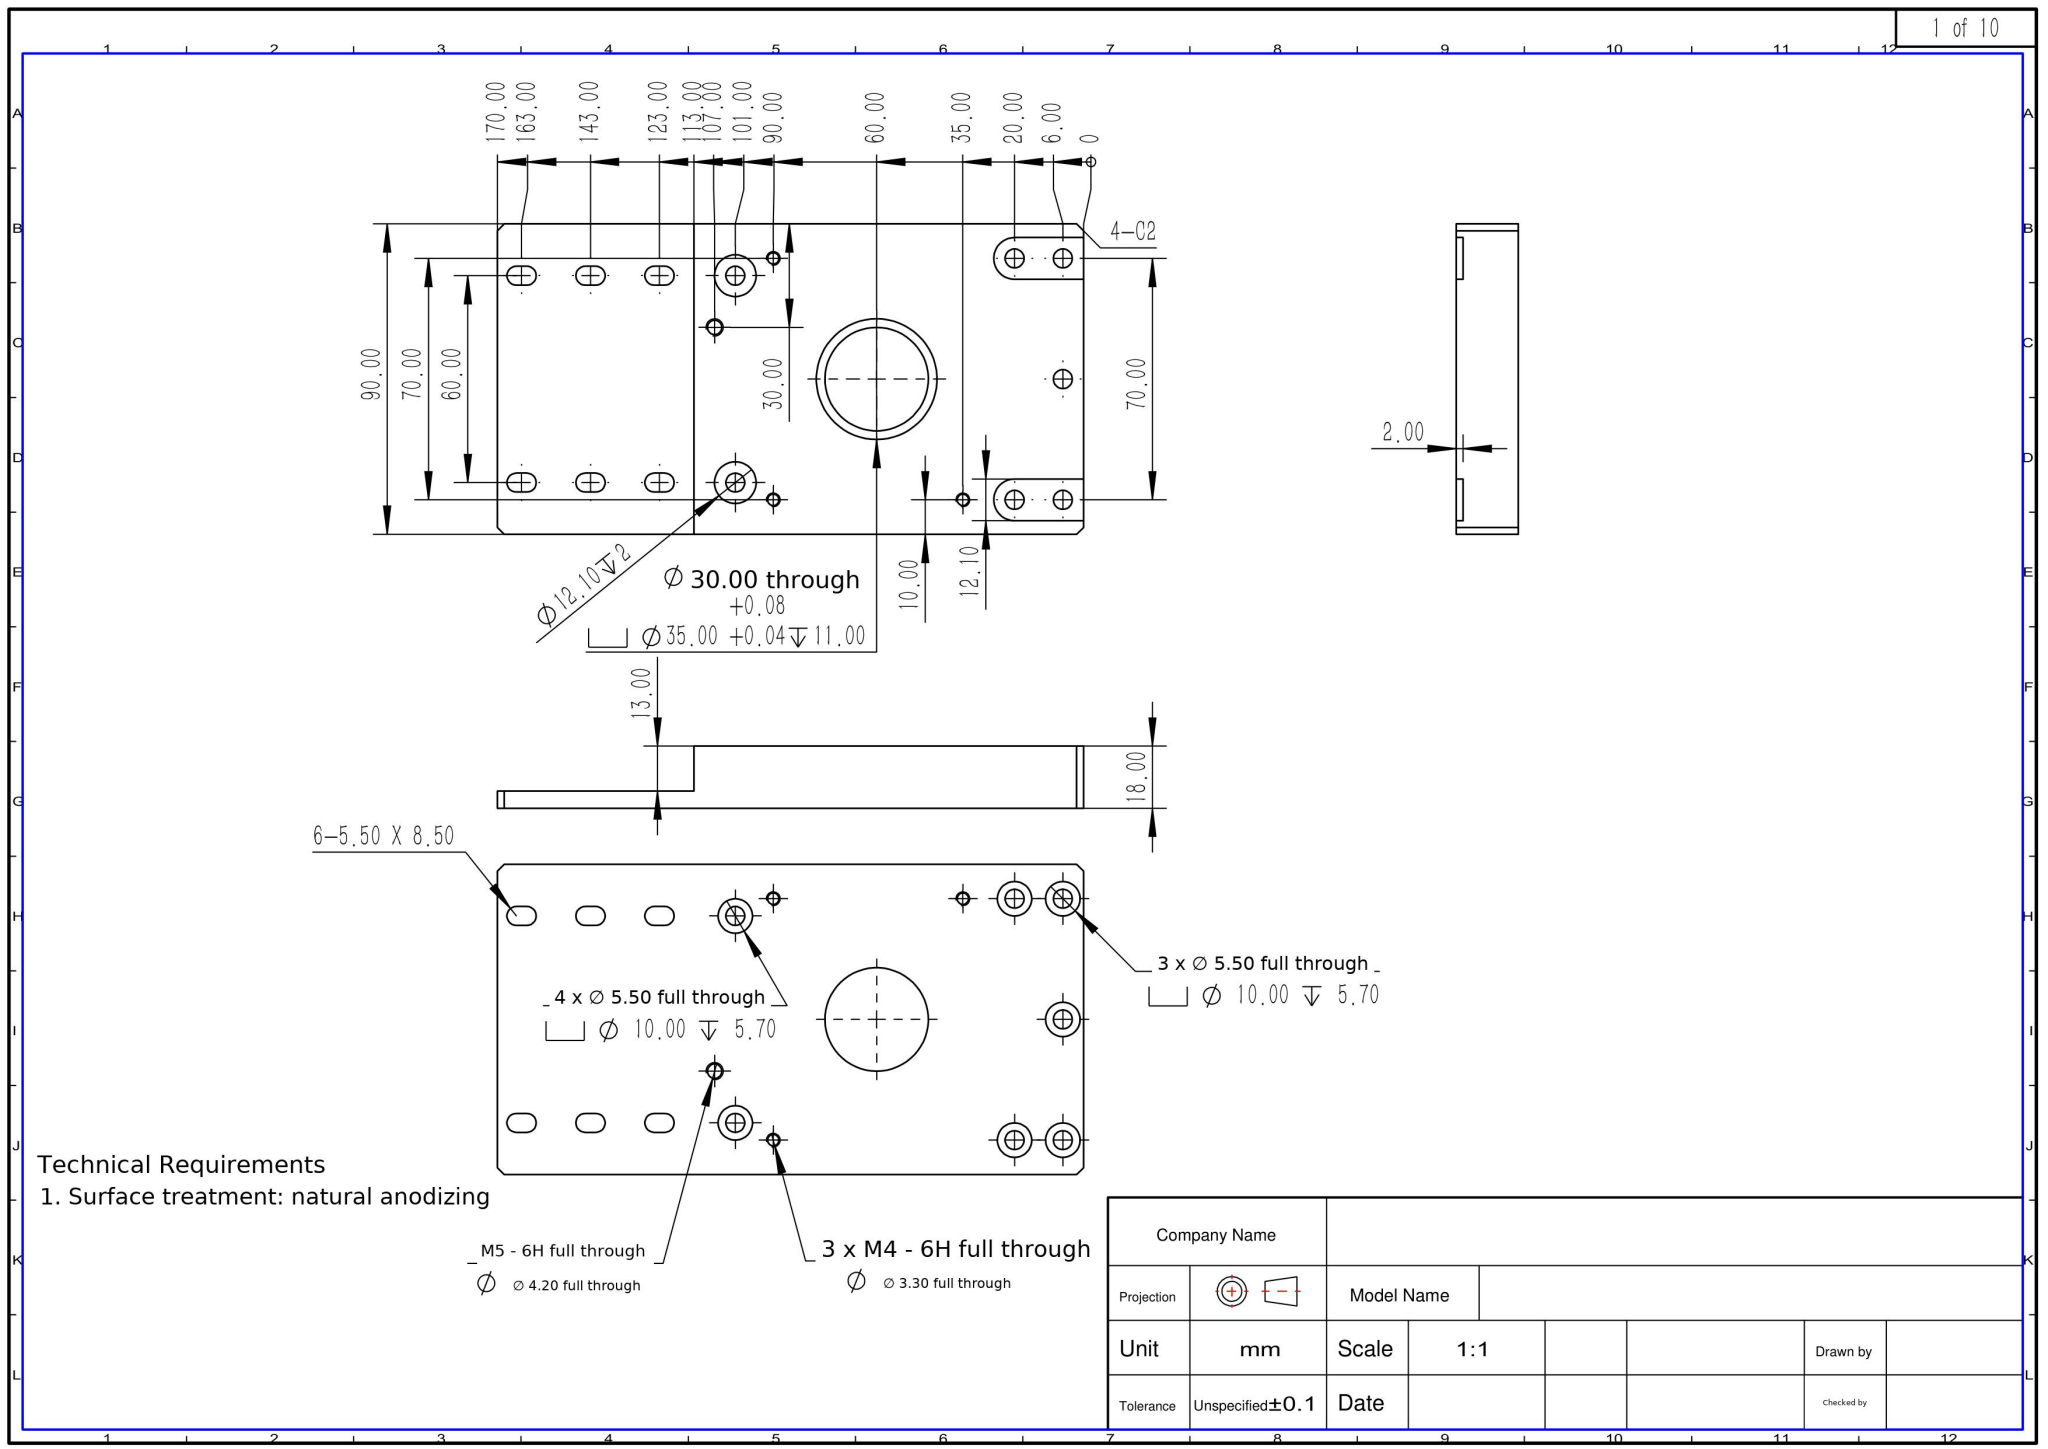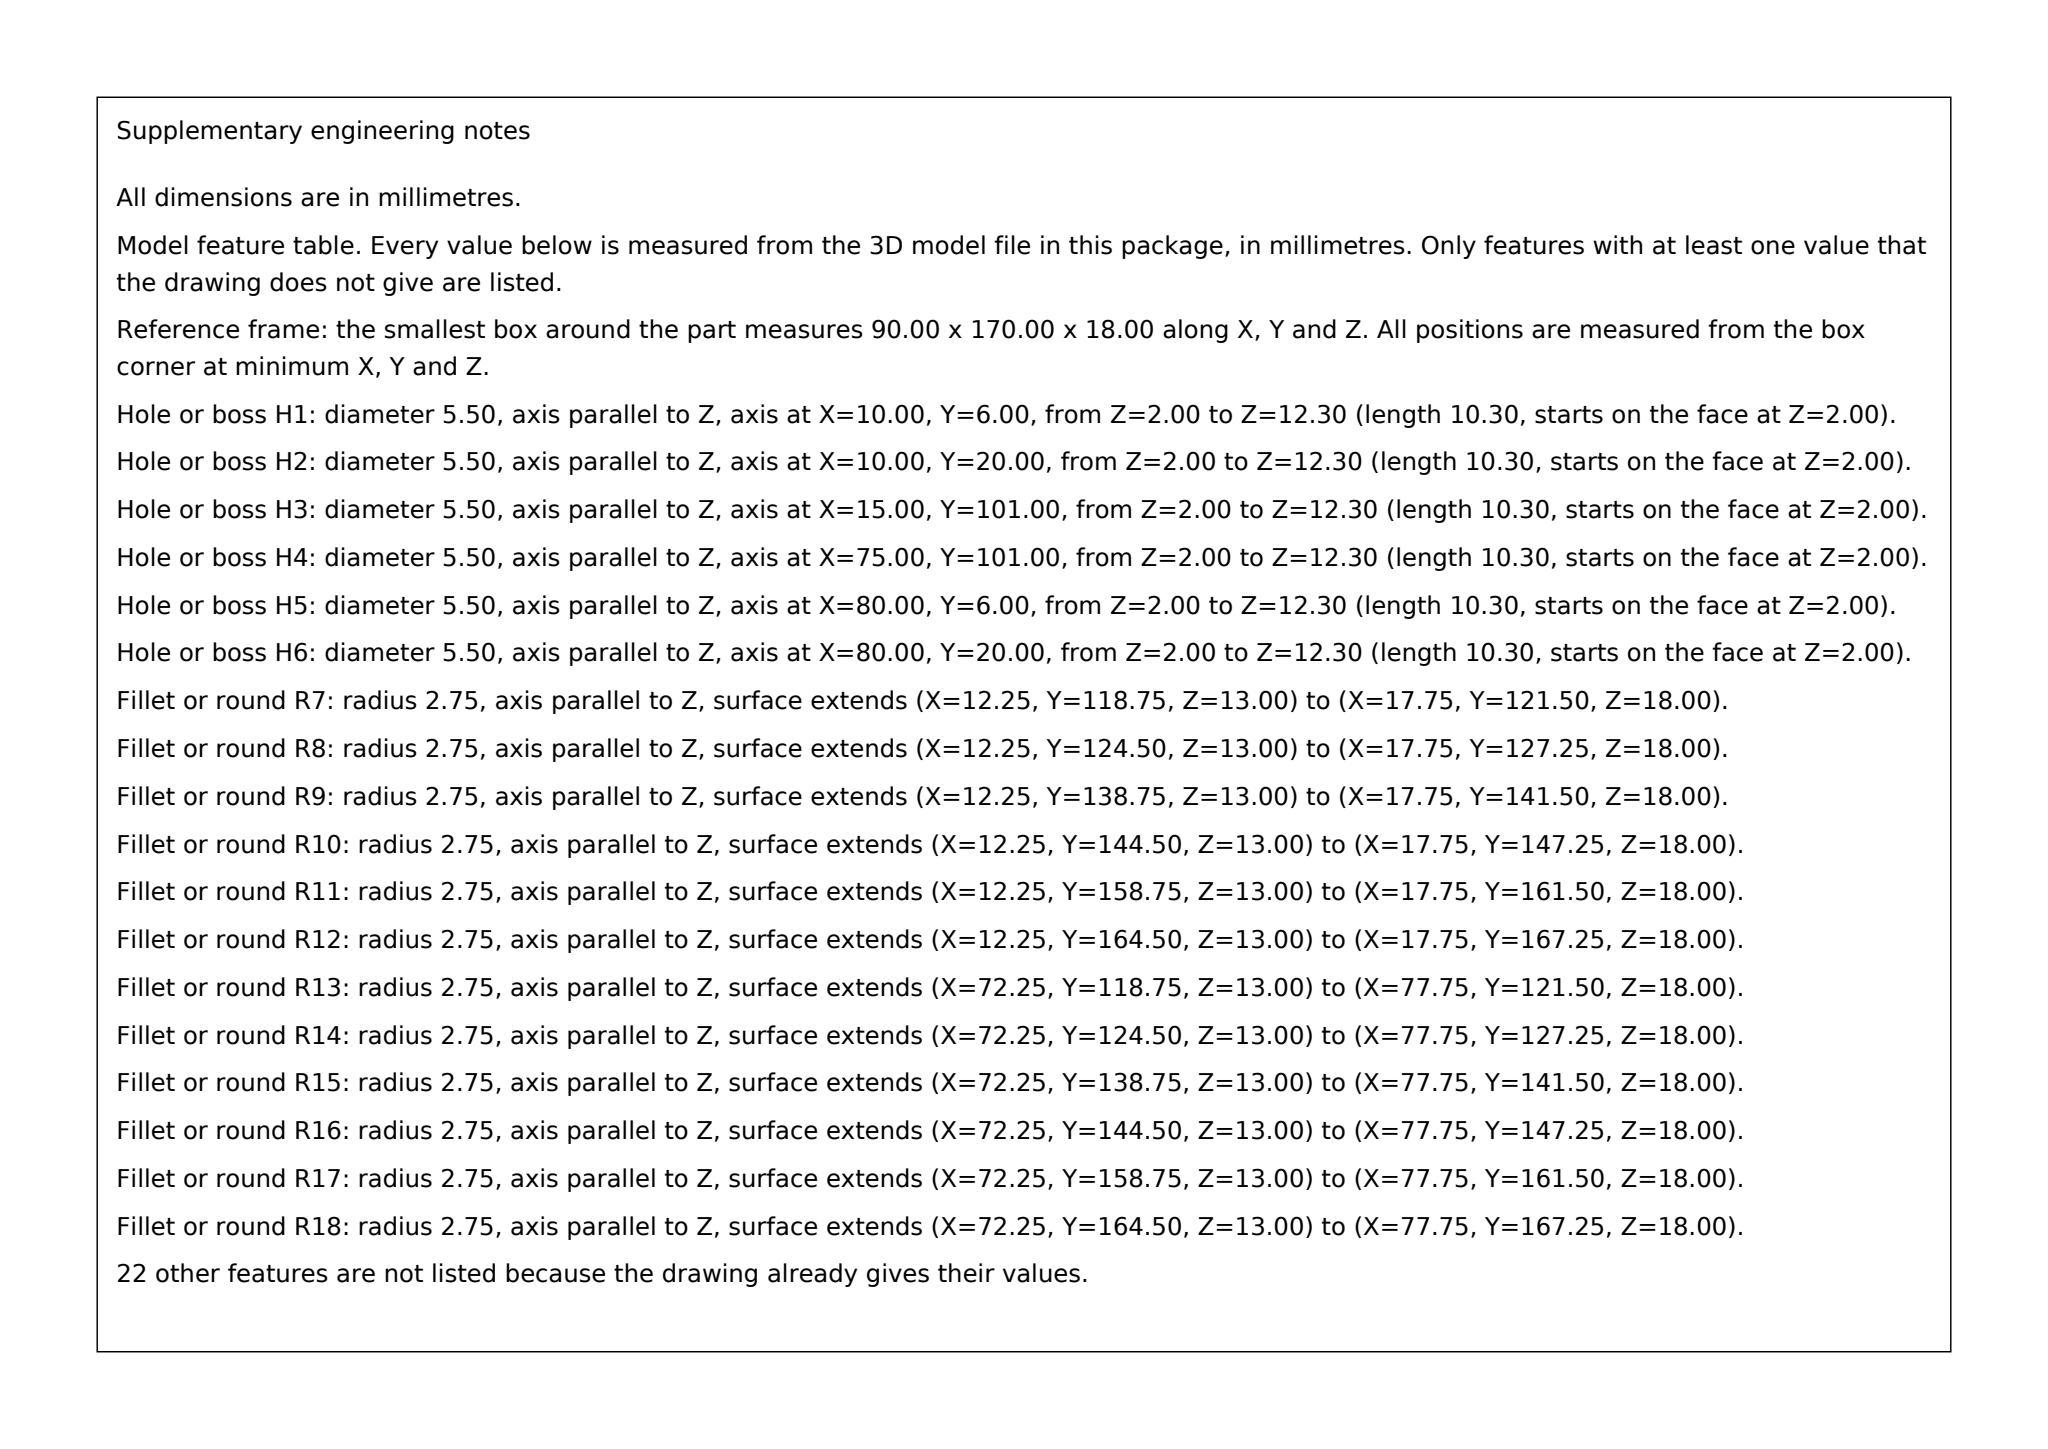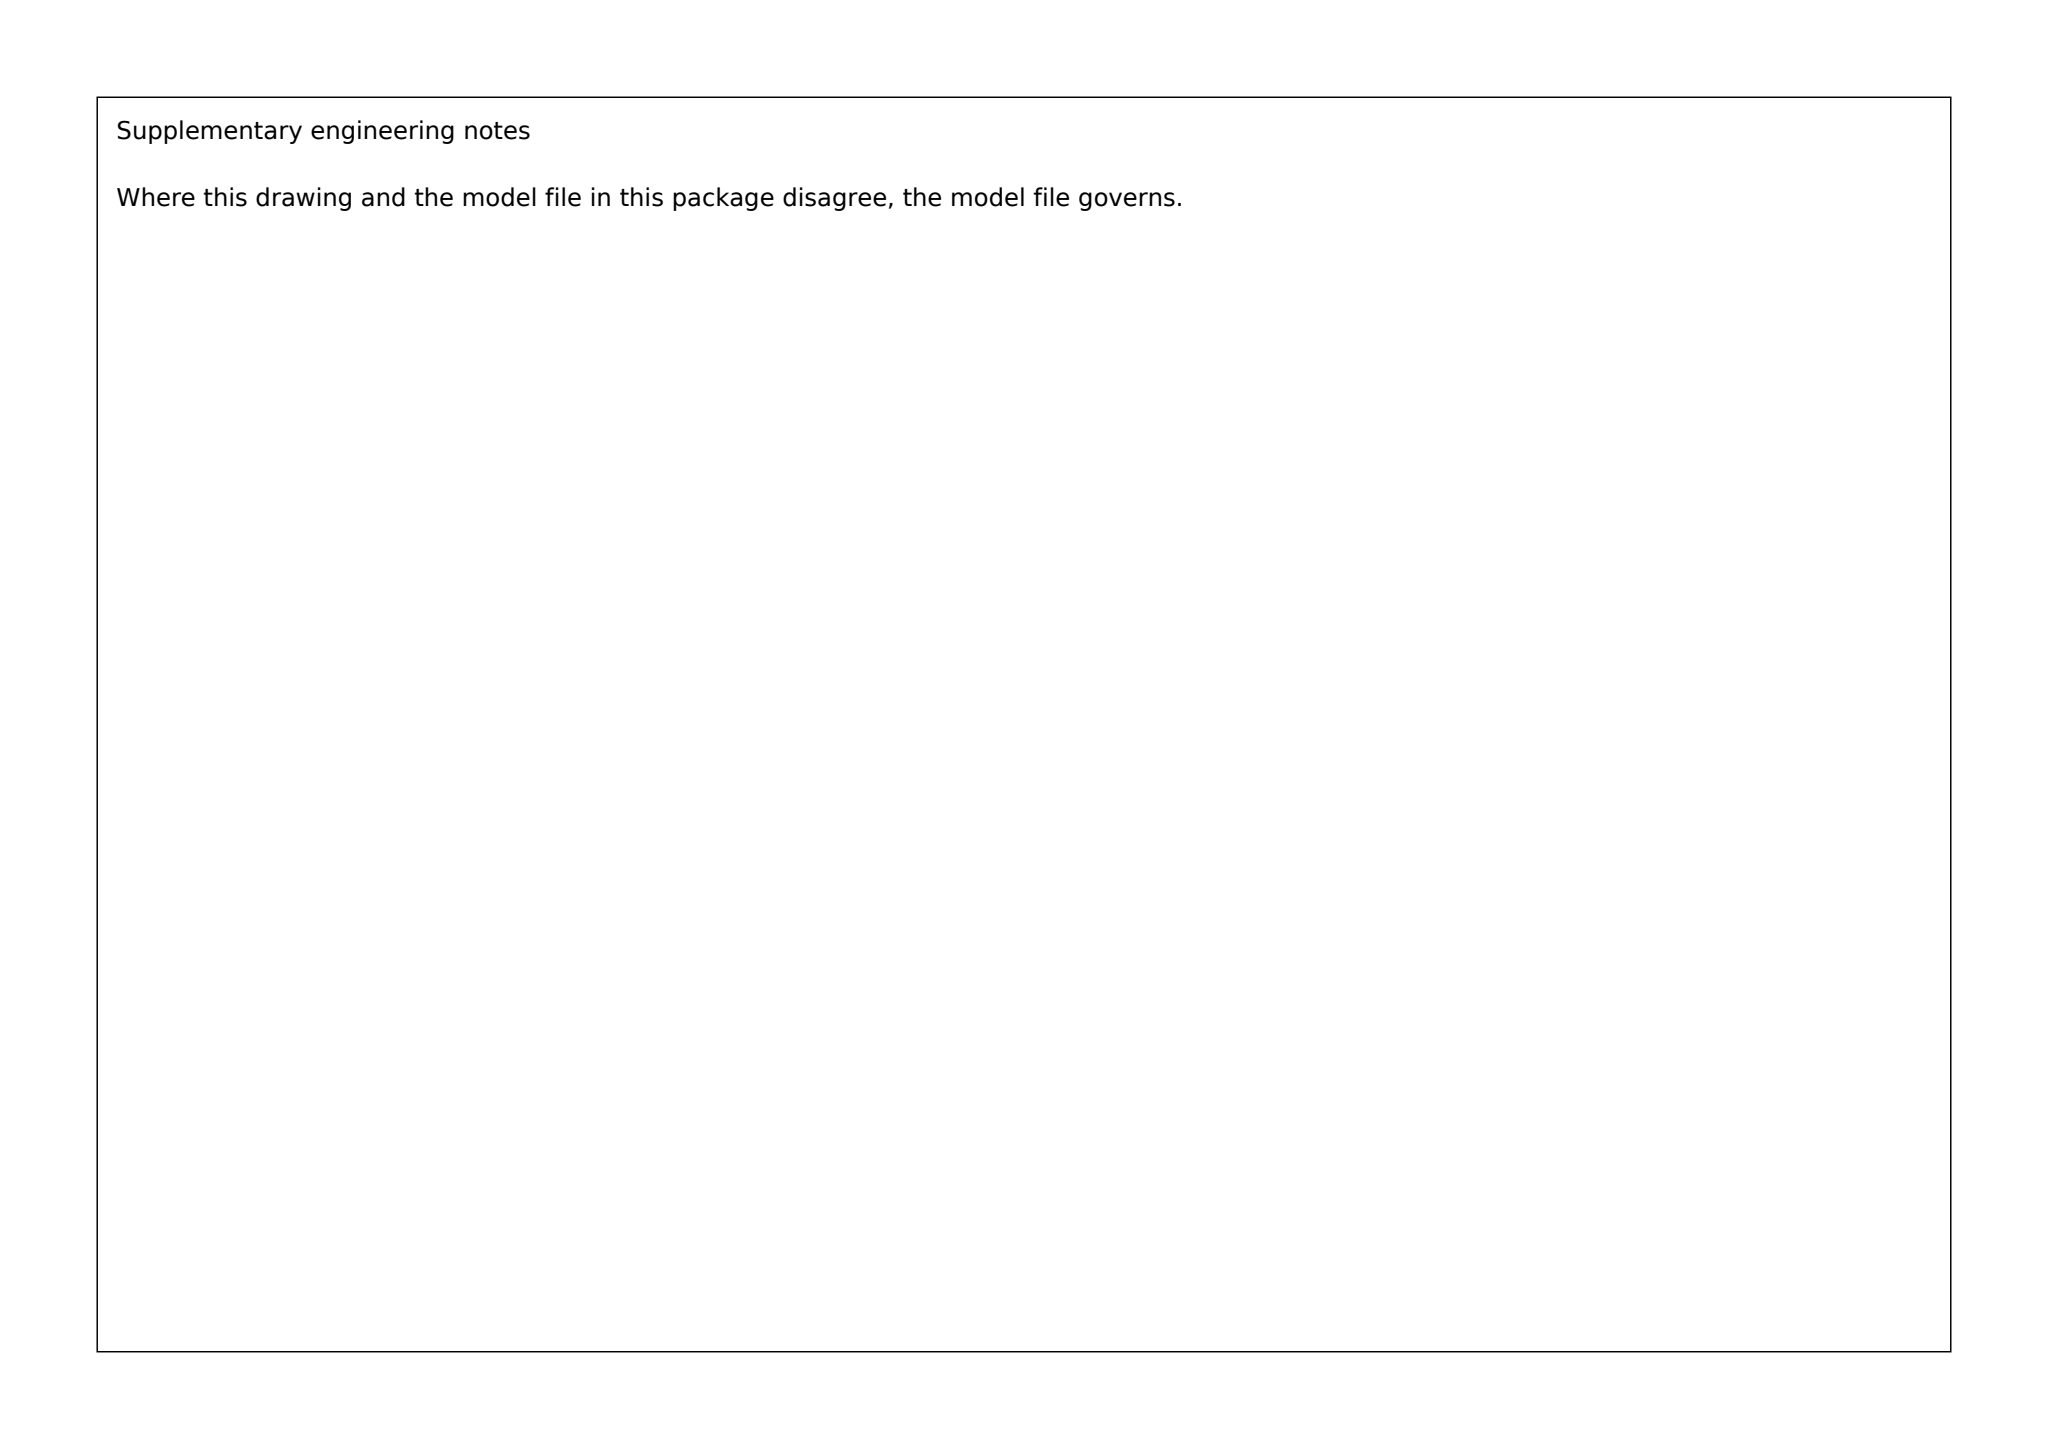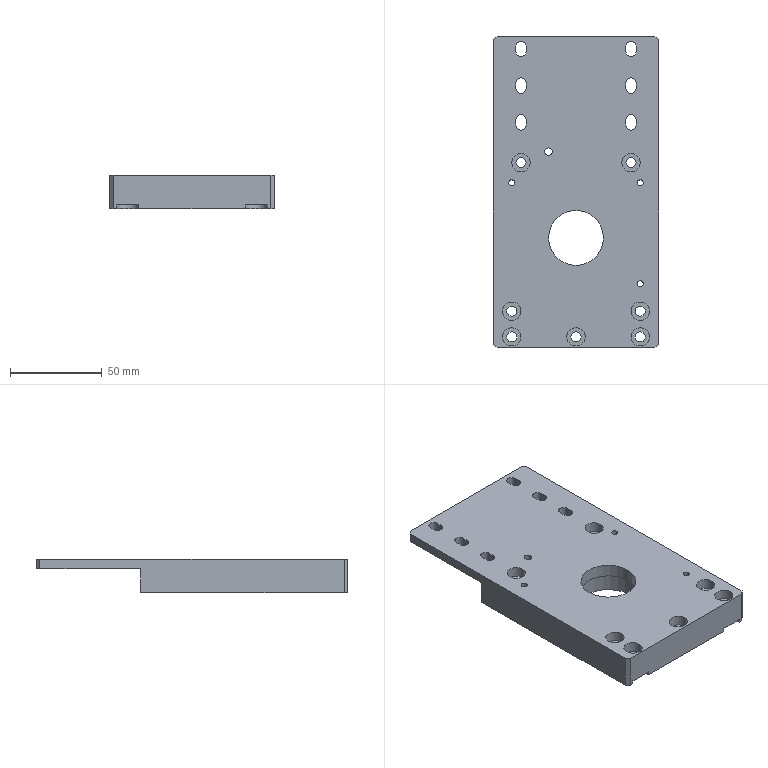Part | SolidWorks | mm | 1 solid | 98 faces | box 90 x 170 x 18 mm | volume 184616 mm3 | cylinder 58 | plane 40 | commonest cylinder face diameters 5.5 x26 10 x14 3.3 x6 12.1 x6 4.2 x2 30 x2 35 x2
build123d program:
from build123d import *

# Parameters (mm, degrees)
SKETCH1_W                                         = 90
SKETCH1_H                                         = 170
BOSS_EXTRUDE1_DEPTH                               = 9
SKETCH2_W                                         = 90
SKETCH2_H                                         = 57
CUT_EXTRUDE1_DEPTH                                = 13
SKETCH3_R                                         = 17.5
CUT_EXTRUDE2_DEPTH                                = 11
SKETCH4_R                                         = 15
CUT_EXTRUDE3_DEPTH                                = 97.804
SKETCH5_R                                         = 6.05
CUT_EXTRUDE4_DEPTH                                = 2
HOLE_SIZE_ACCORDING_TO_TYPE_1_OF_HEXA_D           = 5.5
HOLE_SIZE_ACCORDING_TO_TYPE_1_OF_HEXA_CBORE_D     = 10
HOLE_SIZE_ACCORDING_TO_TYPE_1_OF_HEXA_CBORE_DEPTH = 5.7
CHAMFER1_SIZE                                     = 2
HOLE_SIZE_ACCORDING_TO_TYPE_2_OF_HEXA_D           = 5.5
HOLE_SIZE_ACCORDING_TO_TYPE_2_OF_HEXA_CBORE_D     = 10
HOLE_SIZE_ACCORDING_TO_TYPE_2_OF_HEXA_CBORE_DEPTH = 5.7
M5_TAPPED_HOLE1_D                                 = 4.2
M4_TAPPED_HOLE1_D                                 = 3.3
CUT_EXTRUDE5_DEPTH                                = 98.847


with BuildPart() as part:
    # Sketch1 → Boss-Extrude1 (new, symmetric)
    with BuildSketch(Plane.XY):
        Rectangle(SKETCH1_W, SKETCH1_H)
    extrude(amount=BOSS_EXTRUDE1_DEPTH, both=True)

    # Sketch2 → Cut-Extrude1 (cut)
    with BuildSketch(Plane(origin=(0, 0, -9), x_dir=(-1, 0, 0), z_dir=(0, 0, -1))):
        with Locations((0, 56.5)):
            Rectangle(SKETCH2_W, SKETCH2_H)
    extrude(amount=-CUT_EXTRUDE1_DEPTH, mode=Mode.SUBTRACT)

    # Sketch3 → Cut-Extrude2 (cut)
    with BuildSketch(Plane(origin=(0, 0, -9), x_dir=(-1, 0, 0), z_dir=(0, 0, -1))):
        with Locations((0, -25)):
            Circle(SKETCH3_R)
    extrude(amount=-CUT_EXTRUDE2_DEPTH, mode=Mode.SUBTRACT)

    # Sketch4 → Cut-Extrude3 (cut, through all)
    with BuildSketch(Plane(origin=(0, 0, 2), x_dir=(-1, 0, 0), z_dir=(0, 0, -1))):
        with Locations((0, -25)):
            Circle(SKETCH4_R)
    extrude(amount=-CUT_EXTRUDE3_DEPTH, mode=Mode.SUBTRACT)

    # Sketch5 → Cut-Extrude4 (cut)
    with BuildSketch(Plane(origin=(0, 0, -9), x_dir=(-1, 0, 0), z_dir=(0, 0, -1))):
        with Locations((-30, 16)):
            Circle(SKETCH5_R)
        with Locations((30, 16)):
            Circle(SKETCH5_R)
        with BuildLine():
            Line((-28.95, -65), (-28.95, -85))
            ThreePointArc((-28.95, -85), (-35, -91.05), (-41.05, -85))
            Line((-41.05, -85), (-41.05, -65))
            ThreePointArc((-41.05, -65), (-35, -58.95), (-28.95, -65))
        make_face()
        with BuildLine():
            Line((41.05, -65), (41.05, -85))
            ThreePointArc((41.05, -85), (35, -91.05), (28.95, -85))
            Line((28.95, -85), (28.95, -65))
            ThreePointArc((28.95, -65), (35, -58.95), (41.05, -65))
        make_face()
    extrude(amount=-CUT_EXTRUDE4_DEPTH, mode=Mode.SUBTRACT)

    # Hole Size _ according to_ Type 1 of Hexa (through all)
    with Locations(Plane.XY.offset(9)):
        with Locations((-35, -65), (35, -65), (30, 16), (-30, 16)):
            CounterBoreHole(HOLE_SIZE_ACCORDING_TO_TYPE_1_OF_HEXA_D / 2, HOLE_SIZE_ACCORDING_TO_TYPE_1_OF_HEXA_CBORE_D / 2, HOLE_SIZE_ACCORDING_TO_TYPE_1_OF_HEXA_CBORE_DEPTH)

    # Chamfer1
    chamfer1_edges = [part.edges().sort_by_distance(p)[0] for p in [
        (45, -85, 0),
        (-45, -85, 0),
        (-45, 85, 6.5),
        (45, 85, 6.5),
    ]]
    chamfer(chamfer1_edges, length=CHAMFER1_SIZE)

    # Hole Size _ according to_ Type 2 of Hexa (through all)
    with Locations(Plane.XY.offset(9)):
        with Locations((-35, -79), (0, -79), (35, -79)):
            CounterBoreHole(HOLE_SIZE_ACCORDING_TO_TYPE_2_OF_HEXA_D / 2, HOLE_SIZE_ACCORDING_TO_TYPE_2_OF_HEXA_CBORE_D / 2, HOLE_SIZE_ACCORDING_TO_TYPE_2_OF_HEXA_CBORE_DEPTH)

    # M5 Tapped Hole1 (through all)
    with Locations(Plane.XY.offset(9)):
        with Locations((-15, 22)):
            Hole(M5_TAPPED_HOLE1_D / 2)

    # M4 Tapped Hole1 (through all)
    with Locations(Plane.XY.offset(9)):
        with Locations((35, -50), (-35, 5), (35, 5)):
            Hole(M4_TAPPED_HOLE1_D / 2)

    # Sketch14 → Cut-Extrude5 (cut, through all)
    with BuildSketch(Plane.XY.offset(9)):
        with BuildLine():
            Line((-27.25, 79.5), (-27.25, 76.5))
            ThreePointArc((-27.25, 76.5), (-30, 73.75), (-32.75, 76.5))
            Line((-32.75, 76.5), (-32.75, 79.5))
            ThreePointArc((-32.75, 79.5), (-30, 82.25), (-27.25, 79.5))
        make_face()
        with BuildLine():
            Line((32.75, 79.5), (32.75, 76.5))
            ThreePointArc((32.75, 76.5), (30, 73.75), (27.25, 76.5))
            Line((27.25, 76.5), (27.25, 79.5))
            ThreePointArc((27.25, 79.5), (30, 82.25), (32.75, 79.5))
        make_face()
        with BuildLine():
            Line((-27.25, 59.5), (-27.25, 56.5))
            ThreePointArc((-27.25, 56.5), (-30, 53.75), (-32.75, 56.5))
            Line((-32.75, 56.5), (-32.75, 59.5))
            ThreePointArc((-32.75, 59.5), (-30, 62.25), (-27.25, 59.5))
        make_face()
        with BuildLine():
            Line((32.75, 59.5), (32.75, 56.5))
            ThreePointArc((32.75, 56.5), (30, 53.75), (27.25, 56.5))
            Line((27.25, 56.5), (27.25, 59.5))
            ThreePointArc((27.25, 59.5), (30, 62.25), (32.75, 59.5))
        make_face()
        with BuildLine():
            Line((-27.25, 39.5), (-27.25, 36.5))
            ThreePointArc((-27.25, 36.5), (-30, 33.75), (-32.75, 36.5))
            Line((-32.75, 36.5), (-32.75, 39.5))
            ThreePointArc((-32.75, 39.5), (-30, 42.25), (-27.25, 39.5))
        make_face()
        with BuildLine():
            Line((32.75, 39.5), (32.75, 36.5))
            ThreePointArc((32.75, 36.5), (30, 33.75), (27.25, 36.5))
            Line((27.25, 36.5), (27.25, 39.5))
            ThreePointArc((27.25, 39.5), (30, 42.25), (32.75, 39.5))
        make_face()
    extrude(amount=-CUT_EXTRUDE5_DEPTH, mode=Mode.SUBTRACT)


solid = part.part